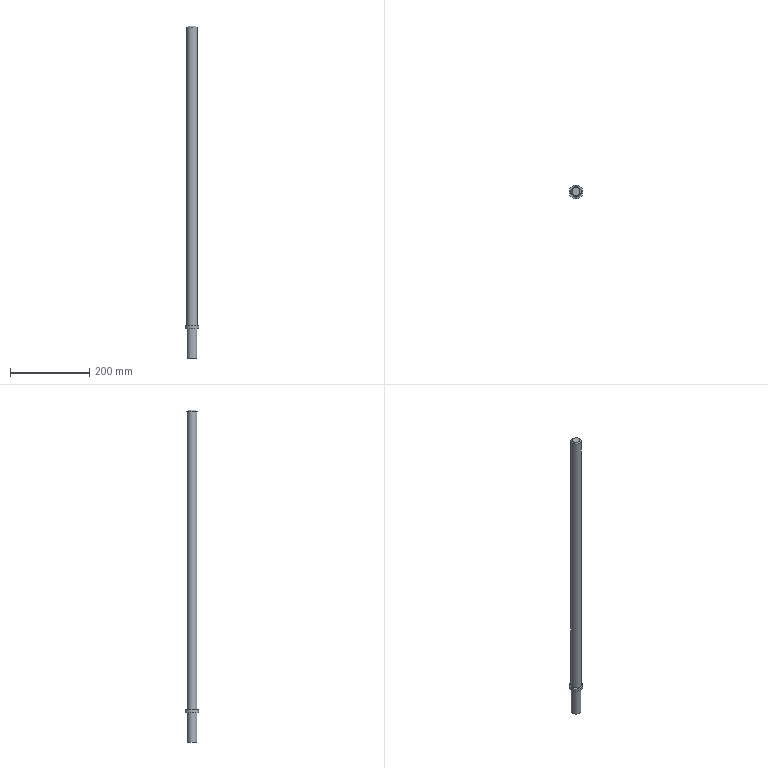Component | NX | SCREW_ROD | 1 solid | 13 faces | box 35 x 35 x 837 mm | volume 443093 mm3 | plane 7 | cylinder 5 | cone 1 | commonest cylinder face diameters 8 x2 25 x1 35 x1 26 x1
STEP:
#1=CARTESIAN_POINT('',(0.,0.,0.));
#2=DIRECTION('',(0.,0.,1.));
#3=DIRECTION('',(1.,0.,0.));
#4=AXIS2_PLACEMENT_3D('',#1,#2,#3);
#5=CARTESIAN_POINT('',(-436.675,308.181,-737.));
#6=VERTEX_POINT('',#5);
#7=CARTESIAN_POINT('',(-424.175,308.181,-737.));
#8=DIRECTION('',(0.,0.,1.));
#9=DIRECTION('',(-1.,0.,0.));
#10=AXIS2_PLACEMENT_3D('',#7,#8,#9);
#11=CIRCLE('',#10,12.5);
#12=CARTESIAN_POINT('',(-424.175,308.181,-737.));
#13=DIRECTION('',(0.,0.,-1.));
#14=DIRECTION('',(-1.,0.,0.));
#15=AXIS2_PLACEMENT_3D('',#12,#13,#14);
#16=PLANE('',#15);
#17=CARTESIAN_POINT('',(12.5,0.));
#18=CARTESIAN_POINT('',(12.5,-21.651));
#19=CARTESIAN_POINT('',(-6.25,-10.825));
#20=CARTESIAN_POINT('',(-25.,-0.));
#21=CARTESIAN_POINT('',(-6.25,10.825));
#22=CARTESIAN_POINT('',(12.5,21.651));
#23=CARTESIAN_POINT('',(12.5,0.));
#24=(BOUNDED_CURVE()B_SPLINE_CURVE(2,(#17,#18,#19,#20,#21,#22,#23),.UNSPECIFIED.,.T.,.F.)B_SPLINE_CURVE_WITH_KNOTS((1,2,2,2,2,1),(-2.094,0.,2.094,4.189,6.283,8.378),.UNSPECIFIED.)CURVE()GEOMETRIC_REPRESENTATION_ITEM()RATIONAL_B_SPLINE_CURVE((1.,0.5,1.,0.5,1.,0.5,1.))REPRESENTATION_ITEM(''));
#25=(GEOMETRIC_REPRESENTATION_CONTEXT(2)PARAMETRIC_REPRESENTATION_CONTEXT()REPRESENTATION_CONTEXT('',''));
#26=DEFINITIONAL_REPRESENTATION('',(#24),#25);
#27=PCURVE('',#16,#26);
#28=CARTESIAN_POINT('',(-424.175,308.181,-707.5));
#29=DIRECTION('',(0.,0.,1.));
#30=DIRECTION('',(1.,0.,0.));
#31=AXIS2_PLACEMENT_3D('',#28,#29,#30);
#32=CYLINDRICAL_SURFACE('',#31,12.5);
#33=CARTESIAN_POINT('',(3.142,-29.5));
#34=DIRECTION('',(1.,0.));
#35=VECTOR('',#34,1.);
#36=LINE('',#33,#35);
#37=(GEOMETRIC_REPRESENTATION_CONTEXT(2)PARAMETRIC_REPRESENTATION_CONTEXT()REPRESENTATION_CONTEXT('',''));
#38=DEFINITIONAL_REPRESENTATION('',(#36),#37);
#39=PCURVE('',#32,#38);
#40=SURFACE_CURVE('',#11,(#27,#39),.PCURVE_S1.);
#41=EDGE_CURVE('',#6,#6,#40,.T.);
#42=ORIENTED_EDGE('',*,*,#41,.F.);
#43=EDGE_LOOP('',(#42));
#44=FACE_BOUND('',#43,.T.);
#45=ADVANCED_FACE('',(#44),#16,.T.);
#46=CARTESIAN_POINT('',(-436.675,308.181,-663.));
#47=VERTEX_POINT('',#46);
#48=CARTESIAN_POINT('',(-424.175,308.181,-663.));
#49=DIRECTION('',(0.,0.,1.));
#50=DIRECTION('',(-1.,0.,0.));
#51=AXIS2_PLACEMENT_3D('',#48,#49,#50);
#52=CIRCLE('',#51,12.5);
#53=CARTESIAN_POINT('',(3.142,44.5));
#54=DIRECTION('',(1.,0.));
#55=VECTOR('',#54,1.);
#56=LINE('',#53,#55);
#57=(GEOMETRIC_REPRESENTATION_CONTEXT(2)PARAMETRIC_REPRESENTATION_CONTEXT()REPRESENTATION_CONTEXT('',''));
#58=DEFINITIONAL_REPRESENTATION('',(#56),#57);
#59=PCURVE('',#32,#58);
#60=CARTESIAN_POINT('',(-424.175,308.181,-663.));
#61=DIRECTION('',(0.,0.,-1.));
#62=DIRECTION('',(-1.,0.,0.));
#63=AXIS2_PLACEMENT_3D('',#60,#61,#62);
#64=PLANE('',#63);
#65=CARTESIAN_POINT('',(12.5,0.));
#66=CARTESIAN_POINT('',(12.5,-21.651));
#67=CARTESIAN_POINT('',(-6.25,-10.825));
#68=CARTESIAN_POINT('',(-25.,-0.));
#69=CARTESIAN_POINT('',(-6.25,10.825));
#70=CARTESIAN_POINT('',(12.5,21.651));
#71=CARTESIAN_POINT('',(12.5,0.));
#72=(BOUNDED_CURVE()B_SPLINE_CURVE(2,(#65,#66,#67,#68,#69,#70,#71),.UNSPECIFIED.,.T.,.F.)B_SPLINE_CURVE_WITH_KNOTS((1,2,2,2,2,1),(-2.094,0.,2.094,4.189,6.283,8.378),.UNSPECIFIED.)CURVE()GEOMETRIC_REPRESENTATION_ITEM()RATIONAL_B_SPLINE_CURVE((1.,0.5,1.,0.5,1.,0.5,1.))REPRESENTATION_ITEM(''));
#73=(GEOMETRIC_REPRESENTATION_CONTEXT(2)PARAMETRIC_REPRESENTATION_CONTEXT()REPRESENTATION_CONTEXT('',''));
#74=DEFINITIONAL_REPRESENTATION('',(#72),#73);
#75=PCURVE('',#64,#74);
#76=SURFACE_CURVE('',#52,(#59,#75),.PCURVE_S1.);
#77=EDGE_CURVE('',#47,#47,#76,.T.);
#78=ORIENTED_EDGE('',*,*,#77,.F.);
#79=CARTESIAN_POINT('',(-436.675,308.181,-737.));
#80=CARTESIAN_POINT('',(-436.675,308.181,-663.));
#81=B_SPLINE_CURVE_WITH_KNOTS('',1,(#79,#80),.UNSPECIFIED.,.F.,.F.,(2,2),(-29.5,44.5),.PIECEWISE_BEZIER_KNOTS.);
#82=CARTESIAN_POINT('',(3.142,0.));
#83=DIRECTION('',(0.,1.));
#84=VECTOR('',#83,1.);
#85=LINE('',#82,#84);
#86=(GEOMETRIC_REPRESENTATION_CONTEXT(2)PARAMETRIC_REPRESENTATION_CONTEXT()REPRESENTATION_CONTEXT('',''));
#87=DEFINITIONAL_REPRESENTATION('',(#85),#86);
#88=PCURVE('',#32,#87);
#89=CARTESIAN_POINT('',(9.425,0.));
#90=DIRECTION('',(0.,1.));
#91=VECTOR('',#90,1.);
#92=LINE('',#89,#91);
#93=(GEOMETRIC_REPRESENTATION_CONTEXT(2)PARAMETRIC_REPRESENTATION_CONTEXT()REPRESENTATION_CONTEXT('',''));
#94=DEFINITIONAL_REPRESENTATION('',(#92),#93);
#95=PCURVE('',#32,#94);
#96=SEAM_CURVE('',#81,(#88,#95),.PCURVE_S1.);
#97=EDGE_CURVE('',#6,#47,#96,.T.);
#98=ORIENTED_EDGE('',*,*,#97,.F.);
#99=ORIENTED_EDGE('',*,*,#41,.T.);
#100=ORIENTED_EDGE('',*,*,#97,.T.);
#101=EDGE_LOOP('',(#78,#98,#99,#100));
#102=FACE_BOUND('',#101,.T.);
#103=CARTESIAN_POINT('',(-420.175,320.024,-689.));
#104=VERTEX_POINT('',#103);
#105=CARTESIAN_POINT('',(-420.175,320.024,-716.));
#106=VERTEX_POINT('',#105);
#107=CARTESIAN_POINT('',(-420.175,320.024,-707.5));
#108=DIRECTION('',(0.,0.,-1.));
#109=VECTOR('',#108,1.);
#110=LINE('',#107,#109);
#111=CARTESIAN_POINT('',(7.528,0.));
#112=DIRECTION('',(0.,-1.));
#113=VECTOR('',#112,1.);
#114=LINE('',#111,#113);
#115=(GEOMETRIC_REPRESENTATION_CONTEXT(2)PARAMETRIC_REPRESENTATION_CONTEXT()REPRESENTATION_CONTEXT('',''));
#116=DEFINITIONAL_REPRESENTATION('',(#114),#115);
#117=PCURVE('',#32,#116);
#118=CARTESIAN_POINT('',(-420.175,308.181,-707.5));
#119=DIRECTION('',(1.,0.,0.));
#120=DIRECTION('',(0.,0.,-1.));
#121=AXIS2_PLACEMENT_3D('',#118,#119,#120);
#122=PLANE('',#121);
#123=CARTESIAN_POINT('',(0.,11.843));
#124=DIRECTION('',(1.,0.));
#125=VECTOR('',#124,1.);
#126=LINE('',#123,#125);
#127=(GEOMETRIC_REPRESENTATION_CONTEXT(2)PARAMETRIC_REPRESENTATION_CONTEXT()REPRESENTATION_CONTEXT('',''));
#128=DEFINITIONAL_REPRESENTATION('',(#126),#127);
#129=PCURVE('',#122,#128);
#130=SURFACE_CURVE('',#110,(#117,#129),.PCURVE_S1.);
#131=EDGE_CURVE('',#104,#106,#130,.T.);
#132=ORIENTED_EDGE('',*,*,#131,.F.);
#133=CARTESIAN_POINT('',(-428.175,320.024,-689.));
#134=VERTEX_POINT('',#133);
#135=CARTESIAN_POINT('',(-420.175,320.024,-689.));
#136=CARTESIAN_POINT('',(-420.175,320.024,-688.565));
#137=CARTESIAN_POINT('',(-420.248,320.049,-688.125));
#138=CARTESIAN_POINT('',(-420.387,320.094,-687.715));
#139=CARTESIAN_POINT('',(-420.526,320.138,-687.306));
#140=CARTESIAN_POINT('',(-420.734,320.201,-686.917));
#141=CARTESIAN_POINT('',(-420.994,320.27,-686.576));
#142=CARTESIAN_POINT('',(-421.262,320.34,-686.223));
#143=CARTESIAN_POINT('',(-421.593,320.418,-685.913));
#144=CARTESIAN_POINT('',(-421.963,320.484,-685.668));
#145=CARTESIAN_POINT('',(-422.341,320.552,-685.417));
#146=CARTESIAN_POINT('',(-422.77,320.61,-685.227));
#147=CARTESIAN_POINT('',(-423.215,320.644,-685.117));
#148=CARTESIAN_POINT('',(-423.527,320.668,-685.04));
#149=CARTESIAN_POINT('',(-423.852,320.681,-685.));
#150=CARTESIAN_POINT('',(-424.175,320.681,-685.));
#151=CARTESIAN_POINT('',(-424.611,320.681,-685.));
#152=CARTESIAN_POINT('',(-425.052,320.657,-685.073));
#153=CARTESIAN_POINT('',(-425.462,320.615,-685.213));
#154=CARTESIAN_POINT('',(-425.872,320.573,-685.352));
#155=CARTESIAN_POINT('',(-426.262,320.511,-685.561));
#156=CARTESIAN_POINT('',(-426.604,320.443,-685.821));
#157=CARTESIAN_POINT('',(-426.955,320.374,-686.09));
#158=CARTESIAN_POINT('',(-427.265,320.296,-686.421));
#159=CARTESIAN_POINT('',(-427.509,320.229,-686.79));
#160=CARTESIAN_POINT('',(-427.76,320.159,-687.168));
#161=CARTESIAN_POINT('',(-427.949,320.099,-687.597));
#162=CARTESIAN_POINT('',(-428.059,320.063,-688.041));
#163=CARTESIAN_POINT('',(-428.136,320.038,-688.353));
#164=CARTESIAN_POINT('',(-428.175,320.024,-688.678));
#165=CARTESIAN_POINT('',(-428.175,320.024,-689.));
#166=B_SPLINE_CURVE_WITH_KNOTS('',3,(#135,#136,#137,#138,#139,#140,#141,#142,#143,#144,#145,#146,#147,#148,#149,#150,#151,#152,#153,#154,#155,#156,#157,#158,#159,#160,#161,#162,#163,#164,#165),.UNSPECIFIED.,.F.,.F.,(4,3,3,3,3,3,3,3,3,3,4),(0.,0.1037,0.2071,0.314,0.4235,0.5,0.6038,0.7074,0.8141,0.9237,1.),.UNSPECIFIED.);
#167=CARTESIAN_POINT('',(7.528,18.5));
#168=CARTESIAN_POINT('',(7.528,18.595));
#169=CARTESIAN_POINT('',(7.529,18.786));
#170=CARTESIAN_POINT('',(7.531,19.073));
#171=CARTESIAN_POINT('',(7.536,19.356));
#172=CARTESIAN_POINT('',(7.542,19.634));
#173=CARTESIAN_POINT('',(7.549,19.904));
#174=CARTESIAN_POINT('',(7.559,20.167));
#175=CARTESIAN_POINT('',(7.569,20.423));
#176=CARTESIAN_POINT('',(7.581,20.668));
#177=CARTESIAN_POINT('',(7.595,20.901));
#178=CARTESIAN_POINT('',(7.609,21.121));
#179=CARTESIAN_POINT('',(7.625,21.329));
#180=CARTESIAN_POINT('',(7.642,21.523));
#181=CARTESIAN_POINT('',(7.661,21.702));
#182=CARTESIAN_POINT('',(7.679,21.864));
#183=CARTESIAN_POINT('',(7.699,22.009));
#184=CARTESIAN_POINT('',(7.72,22.137));
#185=CARTESIAN_POINT('',(7.741,22.247));
#186=CARTESIAN_POINT('',(7.763,22.339));
#187=CARTESIAN_POINT('',(7.785,22.41));
#188=CARTESIAN_POINT('',(7.808,22.462));
#189=CARTESIAN_POINT('',(7.831,22.493));
#190=CARTESIAN_POINT('',(7.854,22.504));
#191=CARTESIAN_POINT('',(7.877,22.493));
#192=CARTESIAN_POINT('',(7.9,22.462));
#193=CARTESIAN_POINT('',(7.923,22.41));
#194=CARTESIAN_POINT('',(7.945,22.339));
#195=CARTESIAN_POINT('',(7.967,22.249));
#196=CARTESIAN_POINT('',(7.988,22.139));
#197=CARTESIAN_POINT('',(8.008,22.011));
#198=CARTESIAN_POINT('',(8.028,21.865));
#199=CARTESIAN_POINT('',(8.047,21.703));
#200=CARTESIAN_POINT('',(8.065,21.525));
#201=CARTESIAN_POINT('',(8.082,21.331));
#202=CARTESIAN_POINT('',(8.098,21.123));
#203=CARTESIAN_POINT('',(8.113,20.902));
#204=CARTESIAN_POINT('',(8.126,20.67));
#205=CARTESIAN_POINT('',(8.139,20.426));
#206=CARTESIAN_POINT('',(8.149,20.171));
#207=CARTESIAN_POINT('',(8.158,19.907));
#208=CARTESIAN_POINT('',(8.166,19.636));
#209=CARTESIAN_POINT('',(8.172,19.36));
#210=CARTESIAN_POINT('',(8.176,19.076));
#211=CARTESIAN_POINT('',(8.179,18.788));
#212=CARTESIAN_POINT('',(8.18,18.596));
#213=CARTESIAN_POINT('',(8.18,18.5));
#214=B_SPLINE_CURVE_WITH_KNOTS('',3,(#167,#168,#169,#170,#171,#172,#173,#174,#175,#176,#177,#178,#179,#180,#181,#182,#183,#184,#185,#186,#187,#188,#189,#190,#191,#192,#193,#194,#195,#196,#197,#198,#199,#200,#201,#202,#203,#204,#205,#206,#207,#208,#209,#210,#211,#212,#213),.UNSPECIFIED.,.F.,.F.,(4,1,1,1,1,1,1,1,1,1,1,1,1,1,1,1,1,1,1,1,1,1,1,1,1,1,1,1,1,1,1,1,1,1,1,1,1,1,1,1,1,1,1,1,4),(0.,0.02273,0.04545,0.06818,0.09091,0.1136,0.1364,0.1591,0.1818,0.2045,0.2273,0.25,0.2727,0.2955,0.3182,0.3409,0.3636,0.3864,0.4091,0.4318,0.4545,0.4773,0.5,0.5227,0.5455,0.5682,0.5909,0.6136,0.6364,0.6591,0.6818,0.7045,0.7273,0.75,0.7727,0.7955,0.8182,0.8409,0.8636,0.8864,0.9091,0.9318,0.9545,0.9773,1.),.QUASI_UNIFORM_KNOTS.);
#215=(GEOMETRIC_REPRESENTATION_CONTEXT(2)PARAMETRIC_REPRESENTATION_CONTEXT()REPRESENTATION_CONTEXT('',''));
#216=DEFINITIONAL_REPRESENTATION('',(#214),#215);
#217=PCURVE('',#32,#216);
#218=CARTESIAN_POINT('',(-424.175,308.181,-689.));
#219=DIRECTION('',(0.,1.,0.));
#220=DIRECTION('',(0.,0.,1.));
#221=AXIS2_PLACEMENT_3D('',#218,#219,#220);
#222=CYLINDRICAL_SURFACE('',#221,4.);
#223=CARTESIAN_POINT('',(1.571,11.843));
#224=CARTESIAN_POINT('',(1.547,11.843));
#225=CARTESIAN_POINT('',(1.499,11.845));
#226=CARTESIAN_POINT('',(1.427,11.856));
#227=CARTESIAN_POINT('',(1.355,11.873));
#228=CARTESIAN_POINT('',(1.284,11.896));
#229=CARTESIAN_POINT('',(1.213,11.925));
#230=CARTESIAN_POINT('',(1.141,11.959));
#231=CARTESIAN_POINT('',(1.07,11.997));
#232=CARTESIAN_POINT('',(0.9985,12.039));
#233=CARTESIAN_POINT('',(0.9276,12.083));
#234=CARTESIAN_POINT('',(0.857,12.129));
#235=CARTESIAN_POINT('',(0.7859,12.175));
#236=CARTESIAN_POINT('',(0.7149,12.222));
#237=CARTESIAN_POINT('',(0.6438,12.268));
#238=CARTESIAN_POINT('',(0.5731,12.311));
#239=CARTESIAN_POINT('',(0.5022,12.351));
#240=CARTESIAN_POINT('',(0.4308,12.388));
#241=CARTESIAN_POINT('',(0.3593,12.421));
#242=CARTESIAN_POINT('',(0.2878,12.449));
#243=CARTESIAN_POINT('',(0.2165,12.471));
#244=CARTESIAN_POINT('',(0.1443,12.488));
#245=CARTESIAN_POINT('',(0.07209,12.498));
#246=CARTESIAN_POINT('',(-0.0001412,12.501));
#247=CARTESIAN_POINT('',(-0.07158,12.498));
#248=CARTESIAN_POINT('',(-0.1436,12.488));
#249=CARTESIAN_POINT('',(-0.2155,12.472));
#250=CARTESIAN_POINT('',(-0.2872,12.449));
#251=CARTESIAN_POINT('',(-0.3583,12.422));
#252=CARTESIAN_POINT('',(-0.4297,12.389));
#253=CARTESIAN_POINT('',(-0.5012,12.352));
#254=CARTESIAN_POINT('',(-0.5725,12.311));
#255=CARTESIAN_POINT('',(-0.6434,12.268));
#256=CARTESIAN_POINT('',(-0.7141,12.223));
#257=CARTESIAN_POINT('',(-0.7851,12.176));
#258=CARTESIAN_POINT('',(-0.8562,12.129));
#259=CARTESIAN_POINT('',(-0.9272,12.083));
#260=CARTESIAN_POINT('',(-0.9979,12.039));
#261=CARTESIAN_POINT('',(-1.069,11.998));
#262=CARTESIAN_POINT('',(-1.14,11.959));
#263=CARTESIAN_POINT('',(-1.212,11.925));
#264=CARTESIAN_POINT('',(-1.283,11.896));
#265=CARTESIAN_POINT('',(-1.354,11.873));
#266=CARTESIAN_POINT('',(-1.427,11.856));
#267=CARTESIAN_POINT('',(-1.499,11.845));
#268=CARTESIAN_POINT('',(-1.547,11.843));
#269=CARTESIAN_POINT('',(-1.571,11.843));
#270=B_SPLINE_CURVE_WITH_KNOTS('',3,(#223,#224,#225,#226,#227,#228,#229,#230,#231,#232,#233,#234,#235,#236,#237,#238,#239,#240,#241,#242,#243,#244,#245,#246,#247,#248,#249,#250,#251,#252,#253,#254,#255,#256,#257,#258,#259,#260,#261,#262,#263,#264,#265,#266,#267,#268,#269),.UNSPECIFIED.,.F.,.F.,(4,1,1,1,1,1,1,1,1,1,1,1,1,1,1,1,1,1,1,1,1,1,1,1,1,1,1,1,1,1,1,1,1,1,1,1,1,1,1,1,1,1,1,1,4),(0.,0.02273,0.04545,0.06818,0.09091,0.1136,0.1364,0.1591,0.1818,0.2045,0.2273,0.25,0.2727,0.2955,0.3182,0.3409,0.3636,0.3864,0.4091,0.4318,0.4545,0.4773,0.5,0.5227,0.5455,0.5682,0.5909,0.6136,0.6364,0.6591,0.6818,0.7045,0.7273,0.75,0.7727,0.7955,0.8182,0.8409,0.8636,0.8864,0.9091,0.9318,0.9545,0.9773,1.),.QUASI_UNIFORM_KNOTS.);
#271=(GEOMETRIC_REPRESENTATION_CONTEXT(2)PARAMETRIC_REPRESENTATION_CONTEXT()REPRESENTATION_CONTEXT('',''));
#272=DEFINITIONAL_REPRESENTATION('',(#270),#271);
#273=PCURVE('',#222,#272);
#274=SURFACE_CURVE('',#166,(#217,#273),.PCURVE_S1.);
#275=EDGE_CURVE('',#104,#134,#274,.T.);
#276=ORIENTED_EDGE('',*,*,#275,.T.);
#277=CARTESIAN_POINT('',(-428.175,320.024,-716.));
#278=VERTEX_POINT('',#277);
#279=CARTESIAN_POINT('',(-428.175,320.024,-707.5));
#280=DIRECTION('',(0.,0.,-1.));
#281=VECTOR('',#280,1.);
#282=LINE('',#279,#281);
#283=CARTESIAN_POINT('',(8.18,0.));
#284=DIRECTION('',(0.,-1.));
#285=VECTOR('',#284,1.);
#286=LINE('',#283,#285);
#287=(GEOMETRIC_REPRESENTATION_CONTEXT(2)PARAMETRIC_REPRESENTATION_CONTEXT()REPRESENTATION_CONTEXT('',''));
#288=DEFINITIONAL_REPRESENTATION('',(#286),#287);
#289=PCURVE('',#32,#288);
#290=CARTESIAN_POINT('',(-428.175,308.181,-707.5));
#291=DIRECTION('',(1.,0.,0.));
#292=DIRECTION('',(0.,0.,-1.));
#293=AXIS2_PLACEMENT_3D('',#290,#291,#292);
#294=PLANE('',#293);
#295=CARTESIAN_POINT('',(0.,11.843));
#296=DIRECTION('',(1.,0.));
#297=VECTOR('',#296,1.);
#298=LINE('',#295,#297);
#299=(GEOMETRIC_REPRESENTATION_CONTEXT(2)PARAMETRIC_REPRESENTATION_CONTEXT()REPRESENTATION_CONTEXT('',''));
#300=DEFINITIONAL_REPRESENTATION('',(#298),#299);
#301=PCURVE('',#294,#300);
#302=SURFACE_CURVE('',#282,(#289,#301),.PCURVE_S1.);
#303=EDGE_CURVE('',#134,#278,#302,.T.);
#304=ORIENTED_EDGE('',*,*,#303,.T.);
#305=CARTESIAN_POINT('',(-428.175,320.024,-716.));
#306=CARTESIAN_POINT('',(-428.175,320.024,-716.435));
#307=CARTESIAN_POINT('',(-428.102,320.049,-716.875));
#308=CARTESIAN_POINT('',(-427.963,320.094,-717.285));
#309=CARTESIAN_POINT('',(-427.824,320.138,-717.694));
#310=CARTESIAN_POINT('',(-427.617,320.201,-718.083));
#311=CARTESIAN_POINT('',(-427.357,320.27,-718.424));
#312=CARTESIAN_POINT('',(-427.088,320.34,-718.777));
#313=CARTESIAN_POINT('',(-426.757,320.418,-719.087));
#314=CARTESIAN_POINT('',(-426.388,320.484,-719.332));
#315=CARTESIAN_POINT('',(-426.01,320.552,-719.583));
#316=CARTESIAN_POINT('',(-425.58,320.61,-719.773));
#317=CARTESIAN_POINT('',(-425.136,320.644,-719.883));
#318=CARTESIAN_POINT('',(-424.823,320.668,-719.96));
#319=CARTESIAN_POINT('',(-424.498,320.681,-720.));
#320=CARTESIAN_POINT('',(-424.175,320.681,-720.));
#321=CARTESIAN_POINT('',(-423.74,320.681,-720.));
#322=CARTESIAN_POINT('',(-423.299,320.657,-719.927));
#323=CARTESIAN_POINT('',(-422.888,320.615,-719.787));
#324=CARTESIAN_POINT('',(-422.478,320.573,-719.648));
#325=CARTESIAN_POINT('',(-422.088,320.511,-719.439));
#326=CARTESIAN_POINT('',(-421.747,320.443,-719.179));
#327=CARTESIAN_POINT('',(-421.396,320.374,-718.91));
#328=CARTESIAN_POINT('',(-421.086,320.296,-718.579));
#329=CARTESIAN_POINT('',(-420.842,320.229,-718.21));
#330=CARTESIAN_POINT('',(-420.591,320.159,-717.832));
#331=CARTESIAN_POINT('',(-420.402,320.099,-717.403));
#332=CARTESIAN_POINT('',(-420.292,320.063,-716.959));
#333=CARTESIAN_POINT('',(-420.215,320.038,-716.647));
#334=CARTESIAN_POINT('',(-420.175,320.024,-716.322));
#335=CARTESIAN_POINT('',(-420.175,320.024,-716.));
#336=B_SPLINE_CURVE_WITH_KNOTS('',3,(#305,#306,#307,#308,#309,#310,#311,#312,#313,#314,#315,#316,#317,#318,#319,#320,#321,#322,#323,#324,#325,#326,#327,#328,#329,#330,#331,#332,#333,#334,#335),.UNSPECIFIED.,.F.,.F.,(4,3,3,3,3,3,3,3,3,3,4),(0.,0.1037,0.2071,0.314,0.4235,0.5,0.6038,0.7074,0.8141,0.9237,1.),.UNSPECIFIED.);
#337=CARTESIAN_POINT('',(8.18,-8.5));
#338=CARTESIAN_POINT('',(8.18,-8.595));
#339=CARTESIAN_POINT('',(8.179,-8.786));
#340=CARTESIAN_POINT('',(8.176,-9.073));
#341=CARTESIAN_POINT('',(8.172,-9.356));
#342=CARTESIAN_POINT('',(8.166,-9.634));
#343=CARTESIAN_POINT('',(8.159,-9.904));
#344=CARTESIAN_POINT('',(8.149,-10.167));
#345=CARTESIAN_POINT('',(8.139,-10.423));
#346=CARTESIAN_POINT('',(8.127,-10.668));
#347=CARTESIAN_POINT('',(8.113,-10.901));
#348=CARTESIAN_POINT('',(8.098,-11.121));
#349=CARTESIAN_POINT('',(8.083,-11.329));
#350=CARTESIAN_POINT('',(8.065,-11.523));
#351=CARTESIAN_POINT('',(8.047,-11.702));
#352=CARTESIAN_POINT('',(8.029,-11.864));
#353=CARTESIAN_POINT('',(8.009,-12.009));
#354=CARTESIAN_POINT('',(7.988,-12.137));
#355=CARTESIAN_POINT('',(7.967,-12.247));
#356=CARTESIAN_POINT('',(7.945,-12.339));
#357=CARTESIAN_POINT('',(7.923,-12.41));
#358=CARTESIAN_POINT('',(7.9,-12.462));
#359=CARTESIAN_POINT('',(7.877,-12.493));
#360=CARTESIAN_POINT('',(7.854,-12.504));
#361=CARTESIAN_POINT('',(7.831,-12.493));
#362=CARTESIAN_POINT('',(7.808,-12.462));
#363=CARTESIAN_POINT('',(7.785,-12.41));
#364=CARTESIAN_POINT('',(7.763,-12.339));
#365=CARTESIAN_POINT('',(7.741,-12.249));
#366=CARTESIAN_POINT('',(7.72,-12.139));
#367=CARTESIAN_POINT('',(7.7,-12.011));
#368=CARTESIAN_POINT('',(7.68,-11.865));
#369=CARTESIAN_POINT('',(7.661,-11.703));
#370=CARTESIAN_POINT('',(7.643,-11.525));
#371=CARTESIAN_POINT('',(7.626,-11.331));
#372=CARTESIAN_POINT('',(7.61,-11.123));
#373=CARTESIAN_POINT('',(7.595,-10.902));
#374=CARTESIAN_POINT('',(7.581,-10.67));
#375=CARTESIAN_POINT('',(7.569,-10.426));
#376=CARTESIAN_POINT('',(7.559,-10.171));
#377=CARTESIAN_POINT('',(7.55,-9.907));
#378=CARTESIAN_POINT('',(7.542,-9.636));
#379=CARTESIAN_POINT('',(7.536,-9.36));
#380=CARTESIAN_POINT('',(7.531,-9.076));
#381=CARTESIAN_POINT('',(7.529,-8.788));
#382=CARTESIAN_POINT('',(7.528,-8.596));
#383=CARTESIAN_POINT('',(7.528,-8.5));
#384=B_SPLINE_CURVE_WITH_KNOTS('',3,(#337,#338,#339,#340,#341,#342,#343,#344,#345,#346,#347,#348,#349,#350,#351,#352,#353,#354,#355,#356,#357,#358,#359,#360,#361,#362,#363,#364,#365,#366,#367,#368,#369,#370,#371,#372,#373,#374,#375,#376,#377,#378,#379,#380,#381,#382,#383),.UNSPECIFIED.,.F.,.F.,(4,1,1,1,1,1,1,1,1,1,1,1,1,1,1,1,1,1,1,1,1,1,1,1,1,1,1,1,1,1,1,1,1,1,1,1,1,1,1,1,1,1,1,1,4),(0.,0.02273,0.04545,0.06818,0.09091,0.1136,0.1364,0.1591,0.1818,0.2045,0.2273,0.25,0.2727,0.2955,0.3182,0.3409,0.3636,0.3864,0.4091,0.4318,0.4545,0.4773,0.5,0.5227,0.5455,0.5682,0.5909,0.6136,0.6364,0.6591,0.6818,0.7045,0.7273,0.75,0.7727,0.7955,0.8182,0.8409,0.8636,0.8864,0.9091,0.9318,0.9545,0.9773,1.),.QUASI_UNIFORM_KNOTS.);
#385=(GEOMETRIC_REPRESENTATION_CONTEXT(2)PARAMETRIC_REPRESENTATION_CONTEXT()REPRESENTATION_CONTEXT('',''));
#386=DEFINITIONAL_REPRESENTATION('',(#384),#385);
#387=PCURVE('',#32,#386);
#388=CARTESIAN_POINT('',(-424.175,308.181,-716.));
#389=DIRECTION('',(0.,-1.,-0.));
#390=DIRECTION('',(0.,0.,-1.));
#391=AXIS2_PLACEMENT_3D('',#388,#389,#390);
#392=CYLINDRICAL_SURFACE('',#391,4.);
#393=CARTESIAN_POINT('',(-1.571,-11.843));
#394=CARTESIAN_POINT('',(-1.547,-11.843));
#395=CARTESIAN_POINT('',(-1.499,-11.845));
#396=CARTESIAN_POINT('',(-1.427,-11.856));
#397=CARTESIAN_POINT('',(-1.355,-11.873));
#398=CARTESIAN_POINT('',(-1.284,-11.896));
#399=CARTESIAN_POINT('',(-1.213,-11.925));
#400=CARTESIAN_POINT('',(-1.141,-11.959));
#401=CARTESIAN_POINT('',(-1.07,-11.997));
#402=CARTESIAN_POINT('',(-0.9985,-12.039));
#403=CARTESIAN_POINT('',(-0.9276,-12.083));
#404=CARTESIAN_POINT('',(-0.857,-12.129));
#405=CARTESIAN_POINT('',(-0.7859,-12.175));
#406=CARTESIAN_POINT('',(-0.7149,-12.222));
#407=CARTESIAN_POINT('',(-0.6438,-12.268));
#408=CARTESIAN_POINT('',(-0.5731,-12.311));
#409=CARTESIAN_POINT('',(-0.5022,-12.351));
#410=CARTESIAN_POINT('',(-0.4308,-12.388));
#411=CARTESIAN_POINT('',(-0.3593,-12.421));
#412=CARTESIAN_POINT('',(-0.2878,-12.449));
#413=CARTESIAN_POINT('',(-0.2165,-12.471));
#414=CARTESIAN_POINT('',(-0.1443,-12.488));
#415=CARTESIAN_POINT('',(-0.07209,-12.498));
#416=CARTESIAN_POINT('',(0.0001412,-12.501));
#417=CARTESIAN_POINT('',(0.07158,-12.498));
#418=CARTESIAN_POINT('',(0.1436,-12.488));
#419=CARTESIAN_POINT('',(0.2155,-12.472));
#420=CARTESIAN_POINT('',(0.2872,-12.449));
#421=CARTESIAN_POINT('',(0.3583,-12.422));
#422=CARTESIAN_POINT('',(0.4297,-12.389));
#423=CARTESIAN_POINT('',(0.5012,-12.352));
#424=CARTESIAN_POINT('',(0.5725,-12.311));
#425=CARTESIAN_POINT('',(0.6434,-12.268));
#426=CARTESIAN_POINT('',(0.7141,-12.223));
#427=CARTESIAN_POINT('',(0.7851,-12.176));
#428=CARTESIAN_POINT('',(0.8562,-12.129));
#429=CARTESIAN_POINT('',(0.9272,-12.083));
#430=CARTESIAN_POINT('',(0.9979,-12.039));
#431=CARTESIAN_POINT('',(1.069,-11.998));
#432=CARTESIAN_POINT('',(1.14,-11.959));
#433=CARTESIAN_POINT('',(1.212,-11.925));
#434=CARTESIAN_POINT('',(1.283,-11.896));
#435=CARTESIAN_POINT('',(1.354,-11.873));
#436=CARTESIAN_POINT('',(1.427,-11.856));
#437=CARTESIAN_POINT('',(1.499,-11.845));
#438=CARTESIAN_POINT('',(1.547,-11.843));
#439=CARTESIAN_POINT('',(1.571,-11.843));
#440=B_SPLINE_CURVE_WITH_KNOTS('',3,(#393,#394,#395,#396,#397,#398,#399,#400,#401,#402,#403,#404,#405,#406,#407,#408,#409,#410,#411,#412,#413,#414,#415,#416,#417,#418,#419,#420,#421,#422,#423,#424,#425,#426,#427,#428,#429,#430,#431,#432,#433,#434,#435,#436,#437,#438,#439),.UNSPECIFIED.,.F.,.F.,(4,1,1,1,1,1,1,1,1,1,1,1,1,1,1,1,1,1,1,1,1,1,1,1,1,1,1,1,1,1,1,1,1,1,1,1,1,1,1,1,1,1,1,1,4),(0.,0.02273,0.04545,0.06818,0.09091,0.1136,0.1364,0.1591,0.1818,0.2045,0.2273,0.25,0.2727,0.2955,0.3182,0.3409,0.3636,0.3864,0.4091,0.4318,0.4545,0.4773,0.5,0.5227,0.5455,0.5682,0.5909,0.6136,0.6364,0.6591,0.6818,0.7045,0.7273,0.75,0.7727,0.7955,0.8182,0.8409,0.8636,0.8864,0.9091,0.9318,0.9545,0.9773,1.),.QUASI_UNIFORM_KNOTS.);
#441=(GEOMETRIC_REPRESENTATION_CONTEXT(2)PARAMETRIC_REPRESENTATION_CONTEXT()REPRESENTATION_CONTEXT('',''));
#442=DEFINITIONAL_REPRESENTATION('',(#440),#441);
#443=PCURVE('',#392,#442);
#444=SURFACE_CURVE('',#336,(#387,#443),.PCURVE_S1.);
#445=EDGE_CURVE('',#278,#106,#444,.T.);
#446=ORIENTED_EDGE('',*,*,#445,.T.);
#447=EDGE_LOOP('',(#132,#276,#304,#446));
#448=FACE_BOUND('',#447,.T.);
#449=ADVANCED_FACE('',(#102,#448),#32,.T.);
#450=CARTESIAN_POINT('',(-411.175,308.181,-656.));
#451=VERTEX_POINT('',#450);
#452=CARTESIAN_POINT('',(-424.175,308.181,-656.));
#453=DIRECTION('',(0.,0.,1.));
#454=DIRECTION('',(1.,0.,0.));
#455=AXIS2_PLACEMENT_3D('',#452,#453,#454);
#456=CIRCLE('',#455,13.);
#457=CARTESIAN_POINT('',(-424.175,308.181,-656.));
#458=DIRECTION('',(0.,0.,1.));
#459=DIRECTION('',(1.,0.,0.));
#460=AXIS2_PLACEMENT_3D('',#457,#458,#459);
#461=PLANE('',#460);
#462=CARTESIAN_POINT('',(0.,0.));
#463=DIRECTION('',(1.,0.));
#464=AXIS2_PLACEMENT_2D('',#462,#463);
#465=CIRCLE('',#464,13.);
#466=(GEOMETRIC_REPRESENTATION_CONTEXT(2)PARAMETRIC_REPRESENTATION_CONTEXT()REPRESENTATION_CONTEXT('',''));
#467=DEFINITIONAL_REPRESENTATION('',(#465),#466);
#468=PCURVE('',#461,#467);
#469=CARTESIAN_POINT('',(-424.175,308.181,100.));
#470=DIRECTION('',(0.,0.,-1.));
#471=DIRECTION('',(-1.,0.,0.));
#472=AXIS2_PLACEMENT_3D('',#469,#470,#471);
#473=CYLINDRICAL_SURFACE('',#472,13.);
#474=CARTESIAN_POINT('',(9.425,756.));
#475=DIRECTION('',(-1.,0.));
#476=VECTOR('',#475,1.);
#477=LINE('',#474,#476);
#478=(GEOMETRIC_REPRESENTATION_CONTEXT(2)PARAMETRIC_REPRESENTATION_CONTEXT()REPRESENTATION_CONTEXT('',''));
#479=DEFINITIONAL_REPRESENTATION('',(#477),#478);
#480=PCURVE('',#473,#479);
#481=SURFACE_CURVE('',#456,(#468,#480),.PCURVE_S1.);
#482=EDGE_CURVE('',#451,#451,#481,.T.);
#483=ORIENTED_EDGE('',*,*,#482,.F.);
#484=EDGE_LOOP('',(#483));
#485=FACE_BOUND('',#484,.T.);
#486=CARTESIAN_POINT('',(-406.675,308.181,-656.));
#487=VERTEX_POINT('',#486);
#488=CARTESIAN_POINT('',(-424.175,308.181,-656.));
#489=DIRECTION('',(0.,0.,-1.));
#490=DIRECTION('',(1.,0.,0.));
#491=AXIS2_PLACEMENT_3D('',#488,#489,#490);
#492=CIRCLE('',#491,17.5);
#493=CARTESIAN_POINT('',(17.5,0.));
#494=CARTESIAN_POINT('',(17.5,-30.311));
#495=CARTESIAN_POINT('',(-8.75,-15.155));
#496=CARTESIAN_POINT('',(-35.,-0.));
#497=CARTESIAN_POINT('',(-8.75,15.155));
#498=CARTESIAN_POINT('',(17.5,30.311));
#499=CARTESIAN_POINT('',(17.5,0.));
#500=(BOUNDED_CURVE()B_SPLINE_CURVE(2,(#493,#494,#495,#496,#497,#498,#499),.UNSPECIFIED.,.T.,.F.)B_SPLINE_CURVE_WITH_KNOTS((1,2,2,2,2,1),(-2.094,0.,2.094,4.189,6.283,8.378),.UNSPECIFIED.)CURVE()GEOMETRIC_REPRESENTATION_ITEM()RATIONAL_B_SPLINE_CURVE((1.,0.5,1.,0.5,1.,0.5,1.))REPRESENTATION_ITEM(''));
#501=(GEOMETRIC_REPRESENTATION_CONTEXT(2)PARAMETRIC_REPRESENTATION_CONTEXT()REPRESENTATION_CONTEXT('',''));
#502=DEFINITIONAL_REPRESENTATION('',(#500),#501);
#503=PCURVE('',#461,#502);
#504=CARTESIAN_POINT('',(-424.175,308.181,-650.));
#505=DIRECTION('',(0.,0.,1.));
#506=DIRECTION('',(1.,0.,0.));
#507=AXIS2_PLACEMENT_3D('',#504,#505,#506);
#508=CYLINDRICAL_SURFACE('',#507,17.5);
#509=CARTESIAN_POINT('',(6.283,-6.));
#510=DIRECTION('',(-1.,0.));
#511=VECTOR('',#510,1.);
#512=LINE('',#509,#511);
#513=(GEOMETRIC_REPRESENTATION_CONTEXT(2)PARAMETRIC_REPRESENTATION_CONTEXT()REPRESENTATION_CONTEXT('',''));
#514=DEFINITIONAL_REPRESENTATION('',(#512),#513);
#515=PCURVE('',#508,#514);
#516=SURFACE_CURVE('',#492,(#503,#515),.PCURVE_S1.);
#517=EDGE_CURVE('',#487,#487,#516,.T.);
#518=ORIENTED_EDGE('',*,*,#517,.F.);
#519=EDGE_LOOP('',(#518));
#520=FACE_BOUND('',#519,.T.);
#521=ADVANCED_FACE('',(#485,#520),#461,.T.);
#522=ORIENTED_EDGE('',*,*,#77,.T.);
#523=EDGE_LOOP('',(#522));
#524=FACE_BOUND('',#523,.T.);
#525=CARTESIAN_POINT('',(-441.675,308.181,-663.));
#526=VERTEX_POINT('',#525);
#527=CARTESIAN_POINT('',(-406.675,308.181,-663.));
#528=VERTEX_POINT('',#527);
#529=CARTESIAN_POINT('',(-424.175,308.181,-663.));
#530=DIRECTION('',(0.,0.,1.));
#531=DIRECTION('',(-1.,0.,0.));
#532=AXIS2_PLACEMENT_3D('',#529,#530,#531);
#533=CIRCLE('',#532,17.5);
#534=CARTESIAN_POINT('',(17.5,0.));
#535=CARTESIAN_POINT('',(17.5,-30.311));
#536=CARTESIAN_POINT('',(-8.75,-15.155));
#537=CARTESIAN_POINT('',(-35.,-0.));
#538=CARTESIAN_POINT('',(-8.75,15.155));
#539=CARTESIAN_POINT('',(17.5,30.311));
#540=CARTESIAN_POINT('',(17.5,0.));
#541=(BOUNDED_CURVE()B_SPLINE_CURVE(2,(#534,#535,#536,#537,#538,#539,#540),.UNSPECIFIED.,.T.,.F.)B_SPLINE_CURVE_WITH_KNOTS((1,2,2,2,2,1),(-2.094,0.,2.094,4.189,6.283,8.378),.UNSPECIFIED.)CURVE()GEOMETRIC_REPRESENTATION_ITEM()RATIONAL_B_SPLINE_CURVE((1.,0.5,1.,0.5,1.,0.5,1.))REPRESENTATION_ITEM(''));
#542=(GEOMETRIC_REPRESENTATION_CONTEXT(2)PARAMETRIC_REPRESENTATION_CONTEXT()REPRESENTATION_CONTEXT('',''));
#543=DEFINITIONAL_REPRESENTATION('',(#541),#542);
#544=PCURVE('',#64,#543);
#545=CARTESIAN_POINT('',(3.142,-13.));
#546=DIRECTION('',(1.,0.));
#547=VECTOR('',#546,1.);
#548=LINE('',#545,#547);
#549=(GEOMETRIC_REPRESENTATION_CONTEXT(2)PARAMETRIC_REPRESENTATION_CONTEXT()REPRESENTATION_CONTEXT('',''));
#550=DEFINITIONAL_REPRESENTATION('',(#548),#549);
#551=PCURVE('',#508,#550);
#552=SURFACE_CURVE('',#533,(#544,#551),.PCURVE_S1.);
#553=EDGE_CURVE('',#526,#528,#552,.T.);
#554=ORIENTED_EDGE('',*,*,#553,.F.);
#555=CARTESIAN_POINT('',(-424.175,308.181,-663.));
#556=DIRECTION('',(0.,0.,1.));
#557=DIRECTION('',(-1.,0.,0.));
#558=AXIS2_PLACEMENT_3D('',#555,#556,#557);
#559=CIRCLE('',#558,17.5);
#560=CARTESIAN_POINT('',(17.5,0.));
#561=CARTESIAN_POINT('',(17.5,-30.311));
#562=CARTESIAN_POINT('',(-8.75,-15.155));
#563=CARTESIAN_POINT('',(-35.,-0.));
#564=CARTESIAN_POINT('',(-8.75,15.155));
#565=CARTESIAN_POINT('',(17.5,30.311));
#566=CARTESIAN_POINT('',(17.5,0.));
#567=(BOUNDED_CURVE()B_SPLINE_CURVE(2,(#560,#561,#562,#563,#564,#565,#566),.UNSPECIFIED.,.T.,.F.)B_SPLINE_CURVE_WITH_KNOTS((1,2,2,2,2,1),(-2.094,0.,2.094,4.189,6.283,8.378),.UNSPECIFIED.)CURVE()GEOMETRIC_REPRESENTATION_ITEM()RATIONAL_B_SPLINE_CURVE((1.,0.5,1.,0.5,1.,0.5,1.))REPRESENTATION_ITEM(''));
#568=(GEOMETRIC_REPRESENTATION_CONTEXT(2)PARAMETRIC_REPRESENTATION_CONTEXT()REPRESENTATION_CONTEXT('',''));
#569=DEFINITIONAL_REPRESENTATION('',(#567),#568);
#570=PCURVE('',#64,#569);
#571=CARTESIAN_POINT('',(-3.142,-13.));
#572=DIRECTION('',(1.,0.));
#573=VECTOR('',#572,1.);
#574=LINE('',#571,#573);
#575=(GEOMETRIC_REPRESENTATION_CONTEXT(2)PARAMETRIC_REPRESENTATION_CONTEXT()REPRESENTATION_CONTEXT('',''));
#576=DEFINITIONAL_REPRESENTATION('',(#574),#575);
#577=PCURVE('',#508,#576);
#578=SURFACE_CURVE('',#559,(#570,#577),.PCURVE_S1.);
#579=EDGE_CURVE('',#528,#526,#578,.T.);
#580=ORIENTED_EDGE('',*,*,#579,.F.);
#581=EDGE_LOOP('',(#554,#580));
#582=FACE_BOUND('',#581,.T.);
#583=ADVANCED_FACE('',(#524,#582),#64,.T.);
#584=ORIENTED_EDGE('',*,*,#517,.T.);
#585=CARTESIAN_POINT('',(-406.675,308.181,-663.));
#586=CARTESIAN_POINT('',(-406.675,308.181,-656.));
#587=B_SPLINE_CURVE_WITH_KNOTS('',1,(#585,#586),.UNSPECIFIED.,.F.,.F.,(2,2),(-13.,-6.),.PIECEWISE_BEZIER_KNOTS.);
#588=CARTESIAN_POINT('',(0.,0.));
#589=DIRECTION('',(0.,1.));
#590=VECTOR('',#589,1.);
#591=LINE('',#588,#590);
#592=(GEOMETRIC_REPRESENTATION_CONTEXT(2)PARAMETRIC_REPRESENTATION_CONTEXT()REPRESENTATION_CONTEXT('',''));
#593=DEFINITIONAL_REPRESENTATION('',(#591),#592);
#594=PCURVE('',#508,#593);
#595=CARTESIAN_POINT('',(6.283,0.));
#596=DIRECTION('',(0.,1.));
#597=VECTOR('',#596,1.);
#598=LINE('',#595,#597);
#599=(GEOMETRIC_REPRESENTATION_CONTEXT(2)PARAMETRIC_REPRESENTATION_CONTEXT()REPRESENTATION_CONTEXT('',''));
#600=DEFINITIONAL_REPRESENTATION('',(#598),#599);
#601=PCURVE('',#508,#600);
#602=SEAM_CURVE('',#587,(#594,#601),.PCURVE_S1.);
#603=EDGE_CURVE('',#528,#487,#602,.T.);
#604=ORIENTED_EDGE('',*,*,#603,.F.);
#605=ORIENTED_EDGE('',*,*,#579,.T.);
#606=ORIENTED_EDGE('',*,*,#553,.T.);
#607=ORIENTED_EDGE('',*,*,#603,.T.);
#608=EDGE_LOOP('',(#584,#604,#605,#606,#607));
#609=FACE_BOUND('',#608,.T.);
#610=ADVANCED_FACE('',(#609),#508,.T.);
#611=CARTESIAN_POINT('',(-411.175,308.181,97.));
#612=VERTEX_POINT('',#611);
#613=CARTESIAN_POINT('',(-424.175,308.181,97.));
#614=DIRECTION('',(0.,0.,-1.));
#615=DIRECTION('',(1.,0.,0.));
#616=AXIS2_PLACEMENT_3D('',#613,#614,#615);
#617=CIRCLE('',#616,13.);
#618=CARTESIAN_POINT('',(3.142,3.));
#619=DIRECTION('',(1.,0.));
#620=VECTOR('',#619,1.);
#621=LINE('',#618,#620);
#622=(GEOMETRIC_REPRESENTATION_CONTEXT(2)PARAMETRIC_REPRESENTATION_CONTEXT()REPRESENTATION_CONTEXT('',''));
#623=DEFINITIONAL_REPRESENTATION('',(#621),#622);
#624=PCURVE('',#473,#623);
#625=CARTESIAN_POINT('',(-424.175,308.181,100.));
#626=DIRECTION('',(0.,0.,-1.));
#627=DIRECTION('',(-1.,0.,0.));
#628=AXIS2_PLACEMENT_3D('',#625,#626,#627);
#629=CONICAL_SURFACE('',#628,10.,0.7854);
#630=CARTESIAN_POINT('',(3.142,3.));
#631=DIRECTION('',(1.,0.));
#632=VECTOR('',#631,1.);
#633=LINE('',#630,#632);
#634=(GEOMETRIC_REPRESENTATION_CONTEXT(2)PARAMETRIC_REPRESENTATION_CONTEXT()REPRESENTATION_CONTEXT('',''));
#635=DEFINITIONAL_REPRESENTATION('',(#633),#634);
#636=PCURVE('',#629,#635);
#637=SURFACE_CURVE('',#617,(#624,#636),.PCURVE_S1.);
#638=EDGE_CURVE('',#612,#612,#637,.T.);
#639=ORIENTED_EDGE('',*,*,#638,.T.);
#640=CARTESIAN_POINT('',(-411.175,308.181,97.));
#641=CARTESIAN_POINT('',(-411.175,308.181,-656.));
#642=B_SPLINE_CURVE_WITH_KNOTS('',1,(#640,#641),.UNSPECIFIED.,.F.,.F.,(2,2),(3.,756.),.PIECEWISE_BEZIER_KNOTS.);
#643=CARTESIAN_POINT('',(9.425,0.));
#644=DIRECTION('',(0.,1.));
#645=VECTOR('',#644,1.);
#646=LINE('',#643,#645);
#647=(GEOMETRIC_REPRESENTATION_CONTEXT(2)PARAMETRIC_REPRESENTATION_CONTEXT()REPRESENTATION_CONTEXT('',''));
#648=DEFINITIONAL_REPRESENTATION('',(#646),#647);
#649=PCURVE('',#473,#648);
#650=CARTESIAN_POINT('',(3.142,0.));
#651=DIRECTION('',(0.,1.));
#652=VECTOR('',#651,1.);
#653=LINE('',#650,#652);
#654=(GEOMETRIC_REPRESENTATION_CONTEXT(2)PARAMETRIC_REPRESENTATION_CONTEXT()REPRESENTATION_CONTEXT('',''));
#655=DEFINITIONAL_REPRESENTATION('',(#653),#654);
#656=PCURVE('',#473,#655);
#657=SEAM_CURVE('',#642,(#649,#656),.PCURVE_S1.);
#658=EDGE_CURVE('',#612,#451,#657,.T.);
#659=ORIENTED_EDGE('',*,*,#658,.T.);
#660=ORIENTED_EDGE('',*,*,#482,.T.);
#661=ORIENTED_EDGE('',*,*,#658,.F.);
#662=EDGE_LOOP('',(#639,#659,#660,#661));
#663=FACE_BOUND('',#662,.T.);
#664=ADVANCED_FACE('',(#663),#473,.T.);
#665=CARTESIAN_POINT('',(-414.175,308.181,100.));
#666=VERTEX_POINT('',#665);
#667=CARTESIAN_POINT('',(-424.175,308.181,100.));
#668=DIRECTION('',(0.,0.,1.));
#669=DIRECTION('',(1.,0.,0.));
#670=AXIS2_PLACEMENT_3D('',#667,#668,#669);
#671=CIRCLE('',#670,10.);
#672=CARTESIAN_POINT('',(-424.175,308.181,100.));
#673=DIRECTION('',(0.,0.,1.));
#674=DIRECTION('',(1.,0.,0.));
#675=AXIS2_PLACEMENT_3D('',#672,#673,#674);
#676=PLANE('',#675);
#677=CARTESIAN_POINT('',(0.,0.));
#678=DIRECTION('',(1.,0.));
#679=AXIS2_PLACEMENT_2D('',#677,#678);
#680=CIRCLE('',#679,10.);
#681=(GEOMETRIC_REPRESENTATION_CONTEXT(2)PARAMETRIC_REPRESENTATION_CONTEXT()REPRESENTATION_CONTEXT('',''));
#682=DEFINITIONAL_REPRESENTATION('',(#680),#681);
#683=PCURVE('',#676,#682);
#684=CARTESIAN_POINT('',(9.425,0.));
#685=DIRECTION('',(-1.,0.));
#686=VECTOR('',#685,1.);
#687=LINE('',#684,#686);
#688=(GEOMETRIC_REPRESENTATION_CONTEXT(2)PARAMETRIC_REPRESENTATION_CONTEXT()REPRESENTATION_CONTEXT('',''));
#689=DEFINITIONAL_REPRESENTATION('',(#687),#688);
#690=PCURVE('',#629,#689);
#691=SURFACE_CURVE('',#671,(#683,#690),.PCURVE_S1.);
#692=EDGE_CURVE('',#666,#666,#691,.T.);
#693=ORIENTED_EDGE('',*,*,#692,.T.);
#694=EDGE_LOOP('',(#693));
#695=FACE_BOUND('',#694,.T.);
#696=ADVANCED_FACE('',(#695),#676,.T.);
#697=ORIENTED_EDGE('',*,*,#638,.F.);
#698=CARTESIAN_POINT('',(-414.175,308.181,100.));
#699=CARTESIAN_POINT('',(-411.175,308.181,97.));
#700=B_SPLINE_CURVE_WITH_KNOTS('',1,(#698,#699),.UNSPECIFIED.,.F.,.F.,(2,2),(0.,4.243),.PIECEWISE_BEZIER_KNOTS.);
#701=CARTESIAN_POINT('',(3.142,0.));
#702=DIRECTION('',(0.,1.));
#703=VECTOR('',#702,1.);
#704=LINE('',#701,#703);
#705=(GEOMETRIC_REPRESENTATION_CONTEXT(2)PARAMETRIC_REPRESENTATION_CONTEXT()REPRESENTATION_CONTEXT('',''));
#706=DEFINITIONAL_REPRESENTATION('',(#704),#705);
#707=PCURVE('',#629,#706);
#708=CARTESIAN_POINT('',(9.425,0.));
#709=DIRECTION('',(0.,1.));
#710=VECTOR('',#709,1.);
#711=LINE('',#708,#710);
#712=(GEOMETRIC_REPRESENTATION_CONTEXT(2)PARAMETRIC_REPRESENTATION_CONTEXT()REPRESENTATION_CONTEXT('',''));
#713=DEFINITIONAL_REPRESENTATION('',(#711),#712);
#714=PCURVE('',#629,#713);
#715=SEAM_CURVE('',#700,(#707,#714),.PCURVE_S1.);
#716=EDGE_CURVE('',#666,#612,#715,.T.);
#717=ORIENTED_EDGE('',*,*,#716,.F.);
#718=ORIENTED_EDGE('',*,*,#692,.F.);
#719=ORIENTED_EDGE('',*,*,#716,.T.);
#720=EDGE_LOOP('',(#697,#717,#718,#719));
#721=FACE_BOUND('',#720,.T.);
#722=ADVANCED_FACE('',(#721),#629,.T.);
#723=CARTESIAN_POINT('',(-420.175,316.681,-716.));
#724=VERTEX_POINT('',#723);
#725=CARTESIAN_POINT('',(-428.175,316.681,-716.));
#726=VERTEX_POINT('',#725);
#727=CARTESIAN_POINT('',(-424.175,316.681,-716.));
#728=DIRECTION('',(0.,1.,0.));
#729=DIRECTION('',(0.,-0.,1.));
#730=AXIS2_PLACEMENT_3D('',#727,#728,#729);
#731=CIRCLE('',#730,4.);
#732=CARTESIAN_POINT('',(-420.175,316.681,-685.));
#733=DIRECTION('',(0.,1.,0.));
#734=DIRECTION('',(0.,-0.,1.));
#735=AXIS2_PLACEMENT_3D('',#732,#733,#734);
#736=PLANE('',#735);
#737=CARTESIAN_POINT('',(-31.,-4.));
#738=DIRECTION('',(1.,0.));
#739=AXIS2_PLACEMENT_2D('',#737,#738);
#740=CIRCLE('',#739,4.);
#741=(GEOMETRIC_REPRESENTATION_CONTEXT(2)PARAMETRIC_REPRESENTATION_CONTEXT()REPRESENTATION_CONTEXT('',''));
#742=DEFINITIONAL_REPRESENTATION('',(#740),#741);
#743=PCURVE('',#736,#742);
#744=CARTESIAN_POINT('',(3.142,-8.5));
#745=DIRECTION('',(-1.,0.));
#746=VECTOR('',#745,1.);
#747=LINE('',#744,#746);
#748=(GEOMETRIC_REPRESENTATION_CONTEXT(2)PARAMETRIC_REPRESENTATION_CONTEXT()REPRESENTATION_CONTEXT('',''));
#749=DEFINITIONAL_REPRESENTATION('',(#747),#748);
#750=PCURVE('',#392,#749);
#751=SURFACE_CURVE('',#731,(#743,#750),.PCURVE_S1.);
#752=EDGE_CURVE('',#724,#726,#751,.T.);
#753=ORIENTED_EDGE('',*,*,#752,.T.);
#754=CARTESIAN_POINT('',(-428.175,316.681,-689.));
#755=VERTEX_POINT('',#754);
#756=CARTESIAN_POINT('',(-428.175,316.681,-685.));
#757=DIRECTION('',(0.,-0.,1.));
#758=VECTOR('',#757,1.);
#759=LINE('',#756,#758);
#760=CARTESIAN_POINT('',(0.,-8.));
#761=DIRECTION('',(1.,0.));
#762=VECTOR('',#761,1.);
#763=LINE('',#760,#762);
#764=(GEOMETRIC_REPRESENTATION_CONTEXT(2)PARAMETRIC_REPRESENTATION_CONTEXT()REPRESENTATION_CONTEXT('',''));
#765=DEFINITIONAL_REPRESENTATION('',(#763),#764);
#766=PCURVE('',#736,#765);
#767=CARTESIAN_POINT('',(-22.5,8.5));
#768=DIRECTION('',(-1.,-0.));
#769=VECTOR('',#768,1.);
#770=LINE('',#767,#769);
#771=(GEOMETRIC_REPRESENTATION_CONTEXT(2)PARAMETRIC_REPRESENTATION_CONTEXT()REPRESENTATION_CONTEXT('',''));
#772=DEFINITIONAL_REPRESENTATION('',(#770),#771);
#773=PCURVE('',#294,#772);
#774=SURFACE_CURVE('',#759,(#766,#773),.PCURVE_S1.);
#775=EDGE_CURVE('',#726,#755,#774,.T.);
#776=ORIENTED_EDGE('',*,*,#775,.T.);
#777=CARTESIAN_POINT('',(-420.175,316.681,-689.));
#778=VERTEX_POINT('',#777);
#779=CARTESIAN_POINT('',(-424.175,316.681,-689.));
#780=DIRECTION('',(0.,1.,0.));
#781=DIRECTION('',(0.,-0.,1.));
#782=AXIS2_PLACEMENT_3D('',#779,#780,#781);
#783=CIRCLE('',#782,4.);
#784=CARTESIAN_POINT('',(-4.,-4.));
#785=DIRECTION('',(1.,0.));
#786=AXIS2_PLACEMENT_2D('',#784,#785);
#787=CIRCLE('',#786,4.);
#788=(GEOMETRIC_REPRESENTATION_CONTEXT(2)PARAMETRIC_REPRESENTATION_CONTEXT()REPRESENTATION_CONTEXT('',''));
#789=DEFINITIONAL_REPRESENTATION('',(#787),#788);
#790=PCURVE('',#736,#789);
#791=CARTESIAN_POINT('',(-6.283,8.5));
#792=DIRECTION('',(1.,0.));
#793=VECTOR('',#792,1.);
#794=LINE('',#791,#793);
#795=(GEOMETRIC_REPRESENTATION_CONTEXT(2)PARAMETRIC_REPRESENTATION_CONTEXT()REPRESENTATION_CONTEXT('',''));
#796=DEFINITIONAL_REPRESENTATION('',(#794),#795);
#797=PCURVE('',#222,#796);
#798=SURFACE_CURVE('',#783,(#790,#797),.PCURVE_S1.);
#799=EDGE_CURVE('',#755,#778,#798,.T.);
#800=ORIENTED_EDGE('',*,*,#799,.T.);
#801=CARTESIAN_POINT('',(-420.175,316.681,-685.));
#802=DIRECTION('',(0.,-0.,1.));
#803=VECTOR('',#802,1.);
#804=LINE('',#801,#803);
#805=CARTESIAN_POINT('',(0.,0.));
#806=DIRECTION('',(1.,0.));
#807=VECTOR('',#806,1.);
#808=LINE('',#805,#807);
#809=(GEOMETRIC_REPRESENTATION_CONTEXT(2)PARAMETRIC_REPRESENTATION_CONTEXT()REPRESENTATION_CONTEXT('',''));
#810=DEFINITIONAL_REPRESENTATION('',(#808),#809);
#811=PCURVE('',#736,#810);
#812=CARTESIAN_POINT('',(-22.5,8.5));
#813=DIRECTION('',(-1.,-0.));
#814=VECTOR('',#813,1.);
#815=LINE('',#812,#814);
#816=(GEOMETRIC_REPRESENTATION_CONTEXT(2)PARAMETRIC_REPRESENTATION_CONTEXT()REPRESENTATION_CONTEXT('',''));
#817=DEFINITIONAL_REPRESENTATION('',(#815),#816);
#818=PCURVE('',#122,#817);
#819=SURFACE_CURVE('',#804,(#811,#818),.PCURVE_S1.);
#820=EDGE_CURVE('',#724,#778,#819,.T.);
#821=ORIENTED_EDGE('',*,*,#820,.F.);
#822=EDGE_LOOP('',(#753,#776,#800,#821));
#823=FACE_BOUND('',#822,.T.);
#824=ADVANCED_FACE('',(#823),#736,.T.);
#825=ORIENTED_EDGE('',*,*,#131,.T.);
#826=CARTESIAN_POINT('',(-420.175,308.181,-716.));
#827=DIRECTION('',(0.,-1.,-0.));
#828=VECTOR('',#827,1.);
#829=LINE('',#826,#828);
#830=CARTESIAN_POINT('',(8.5,0.));
#831=DIRECTION('',(0.,-1.));
#832=VECTOR('',#831,1.);
#833=LINE('',#830,#832);
#834=(GEOMETRIC_REPRESENTATION_CONTEXT(2)PARAMETRIC_REPRESENTATION_CONTEXT()REPRESENTATION_CONTEXT('',''));
#835=DEFINITIONAL_REPRESENTATION('',(#833),#834);
#836=PCURVE('',#122,#835);
#837=CARTESIAN_POINT('',(1.571,0.));
#838=DIRECTION('',(0.,1.));
#839=VECTOR('',#838,1.);
#840=LINE('',#837,#839);
#841=(GEOMETRIC_REPRESENTATION_CONTEXT(2)PARAMETRIC_REPRESENTATION_CONTEXT()REPRESENTATION_CONTEXT('',''));
#842=DEFINITIONAL_REPRESENTATION('',(#840),#841);
#843=PCURVE('',#392,#842);
#844=SURFACE_CURVE('',#829,(#836,#843),.PCURVE_S1.);
#845=EDGE_CURVE('',#106,#724,#844,.T.);
#846=ORIENTED_EDGE('',*,*,#845,.T.);
#847=ORIENTED_EDGE('',*,*,#820,.T.);
#848=CARTESIAN_POINT('',(-420.175,308.181,-689.));
#849=DIRECTION('',(0.,1.,0.));
#850=VECTOR('',#849,1.);
#851=LINE('',#848,#850);
#852=CARTESIAN_POINT('',(-18.5,0.));
#853=DIRECTION('',(0.,1.));
#854=VECTOR('',#853,1.);
#855=LINE('',#852,#854);
#856=(GEOMETRIC_REPRESENTATION_CONTEXT(2)PARAMETRIC_REPRESENTATION_CONTEXT()REPRESENTATION_CONTEXT('',''));
#857=DEFINITIONAL_REPRESENTATION('',(#855),#856);
#858=PCURVE('',#122,#857);
#859=CARTESIAN_POINT('',(1.571,0.));
#860=DIRECTION('',(0.,1.));
#861=VECTOR('',#860,1.);
#862=LINE('',#859,#861);
#863=(GEOMETRIC_REPRESENTATION_CONTEXT(2)PARAMETRIC_REPRESENTATION_CONTEXT()REPRESENTATION_CONTEXT('',''));
#864=DEFINITIONAL_REPRESENTATION('',(#862),#863);
#865=PCURVE('',#222,#864);
#866=SURFACE_CURVE('',#851,(#858,#865),.PCURVE_S1.);
#867=EDGE_CURVE('',#778,#104,#866,.T.);
#868=ORIENTED_EDGE('',*,*,#867,.T.);
#869=EDGE_LOOP('',(#825,#846,#847,#868));
#870=FACE_BOUND('',#869,.T.);
#871=ADVANCED_FACE('',(#870),#122,.F.);
#872=ORIENTED_EDGE('',*,*,#775,.F.);
#873=CARTESIAN_POINT('',(-428.175,320.024,-716.));
#874=DIRECTION('',(0.,1.,0.));
#875=VECTOR('',#874,1.);
#876=LINE('',#873,#875);
#877=CARTESIAN_POINT('',(8.5,11.843));
#878=DIRECTION('',(-0.,1.));
#879=VECTOR('',#878,1.);
#880=LINE('',#877,#879);
#881=(GEOMETRIC_REPRESENTATION_CONTEXT(2)PARAMETRIC_REPRESENTATION_CONTEXT()REPRESENTATION_CONTEXT('',''));
#882=DEFINITIONAL_REPRESENTATION('',(#880),#881);
#883=PCURVE('',#294,#882);
#884=CARTESIAN_POINT('',(-1.571,-11.843));
#885=DIRECTION('',(0.,-1.));
#886=VECTOR('',#885,1.);
#887=LINE('',#884,#886);
#888=(GEOMETRIC_REPRESENTATION_CONTEXT(2)PARAMETRIC_REPRESENTATION_CONTEXT()REPRESENTATION_CONTEXT('',''));
#889=DEFINITIONAL_REPRESENTATION('',(#887),#888);
#890=PCURVE('',#392,#889);
#891=SURFACE_CURVE('',#876,(#883,#890),.PCURVE_S1.);
#892=EDGE_CURVE('',#726,#278,#891,.T.);
#893=ORIENTED_EDGE('',*,*,#892,.T.);
#894=ORIENTED_EDGE('',*,*,#303,.F.);
#895=CARTESIAN_POINT('',(-428.175,316.681,-689.));
#896=DIRECTION('',(0.,-1.,0.));
#897=VECTOR('',#896,1.);
#898=LINE('',#895,#897);
#899=CARTESIAN_POINT('',(-18.5,8.5));
#900=DIRECTION('',(0.,-1.));
#901=VECTOR('',#900,1.);
#902=LINE('',#899,#901);
#903=(GEOMETRIC_REPRESENTATION_CONTEXT(2)PARAMETRIC_REPRESENTATION_CONTEXT()REPRESENTATION_CONTEXT('',''));
#904=DEFINITIONAL_REPRESENTATION('',(#902),#903);
#905=PCURVE('',#294,#904);
#906=CARTESIAN_POINT('',(-1.571,8.5));
#907=DIRECTION('',(0.,-1.));
#908=VECTOR('',#907,1.);
#909=LINE('',#906,#908);
#910=(GEOMETRIC_REPRESENTATION_CONTEXT(2)PARAMETRIC_REPRESENTATION_CONTEXT()REPRESENTATION_CONTEXT('',''));
#911=DEFINITIONAL_REPRESENTATION('',(#909),#910);
#912=PCURVE('',#222,#911);
#913=SURFACE_CURVE('',#898,(#905,#912),.PCURVE_S1.);
#914=EDGE_CURVE('',#134,#755,#913,.T.);
#915=ORIENTED_EDGE('',*,*,#914,.T.);
#916=EDGE_LOOP('',(#872,#893,#894,#915));
#917=FACE_BOUND('',#916,.T.);
#918=ADVANCED_FACE('',(#917),#294,.T.);
#919=ORIENTED_EDGE('',*,*,#752,.T.);
#920=ORIENTED_EDGE('',*,*,#892,.T.);
#921=ORIENTED_EDGE('',*,*,#445,.T.);
#922=ORIENTED_EDGE('',*,*,#845,.T.);
#923=EDGE_LOOP('',(#919,#920,#921,#922));
#924=FACE_BOUND('',#923,.F.);
#925=ADVANCED_FACE('',(#924),#392,.F.);
#926=ORIENTED_EDGE('',*,*,#275,.T.);
#927=ORIENTED_EDGE('',*,*,#914,.T.);
#928=ORIENTED_EDGE('',*,*,#799,.T.);
#929=ORIENTED_EDGE('',*,*,#867,.T.);
#930=EDGE_LOOP('',(#926,#927,#928,#929));
#931=FACE_BOUND('',#930,.F.);
#932=ADVANCED_FACE('',(#931),#222,.F.);
#933=CLOSED_SHELL('',(#45,#449,#521,#583,#610,#664,#696,#722,#824,#871,#918,#925,#932));
#934=MANIFOLD_SOLID_BREP('',#933);
#935=(LENGTH_UNIT()NAMED_UNIT(*)SI_UNIT(.MILLI.,.METRE.));
#936=UNCERTAINTY_MEASURE_WITH_UNIT(LENGTH_MEASURE(0.0001),#935,'','');
#937=(NAMED_UNIT(*)PLANE_ANGLE_UNIT()SI_UNIT($,.RADIAN.));
#938=(NAMED_UNIT(*)SI_UNIT($,.STERADIAN.)SOLID_ANGLE_UNIT());
#939=(GEOMETRIC_REPRESENTATION_CONTEXT(3)GLOBAL_UNCERTAINTY_ASSIGNED_CONTEXT((#936))GLOBAL_UNIT_ASSIGNED_CONTEXT((#935,#937,#938))REPRESENTATION_CONTEXT('',''));
#940=ADVANCED_BREP_SHAPE_REPRESENTATION('',(#4,#934),#939);